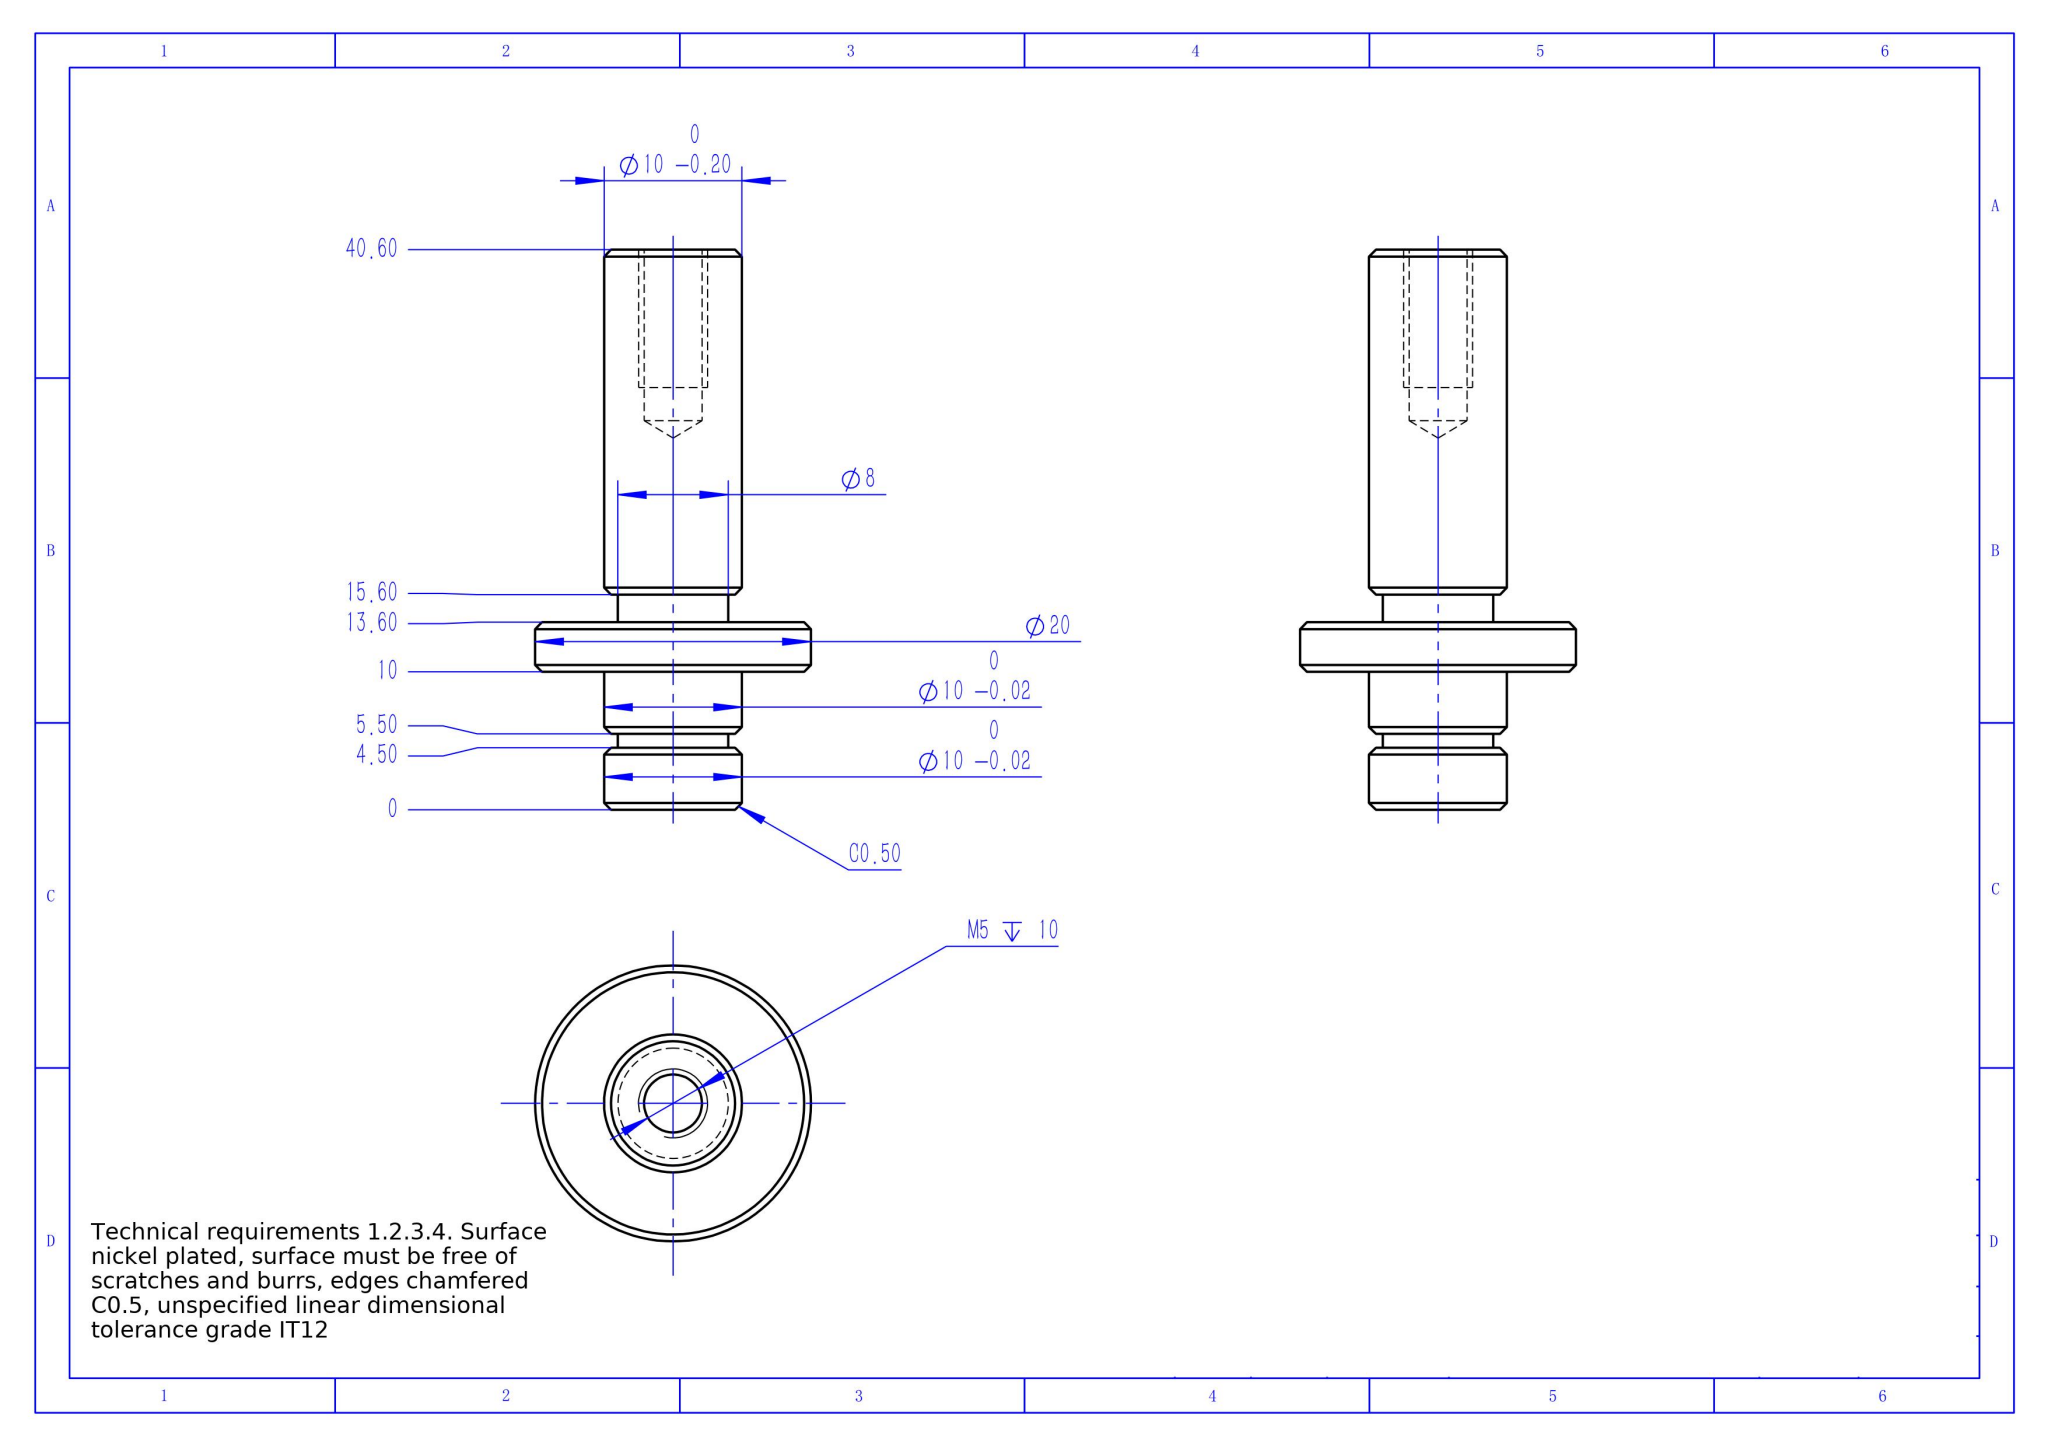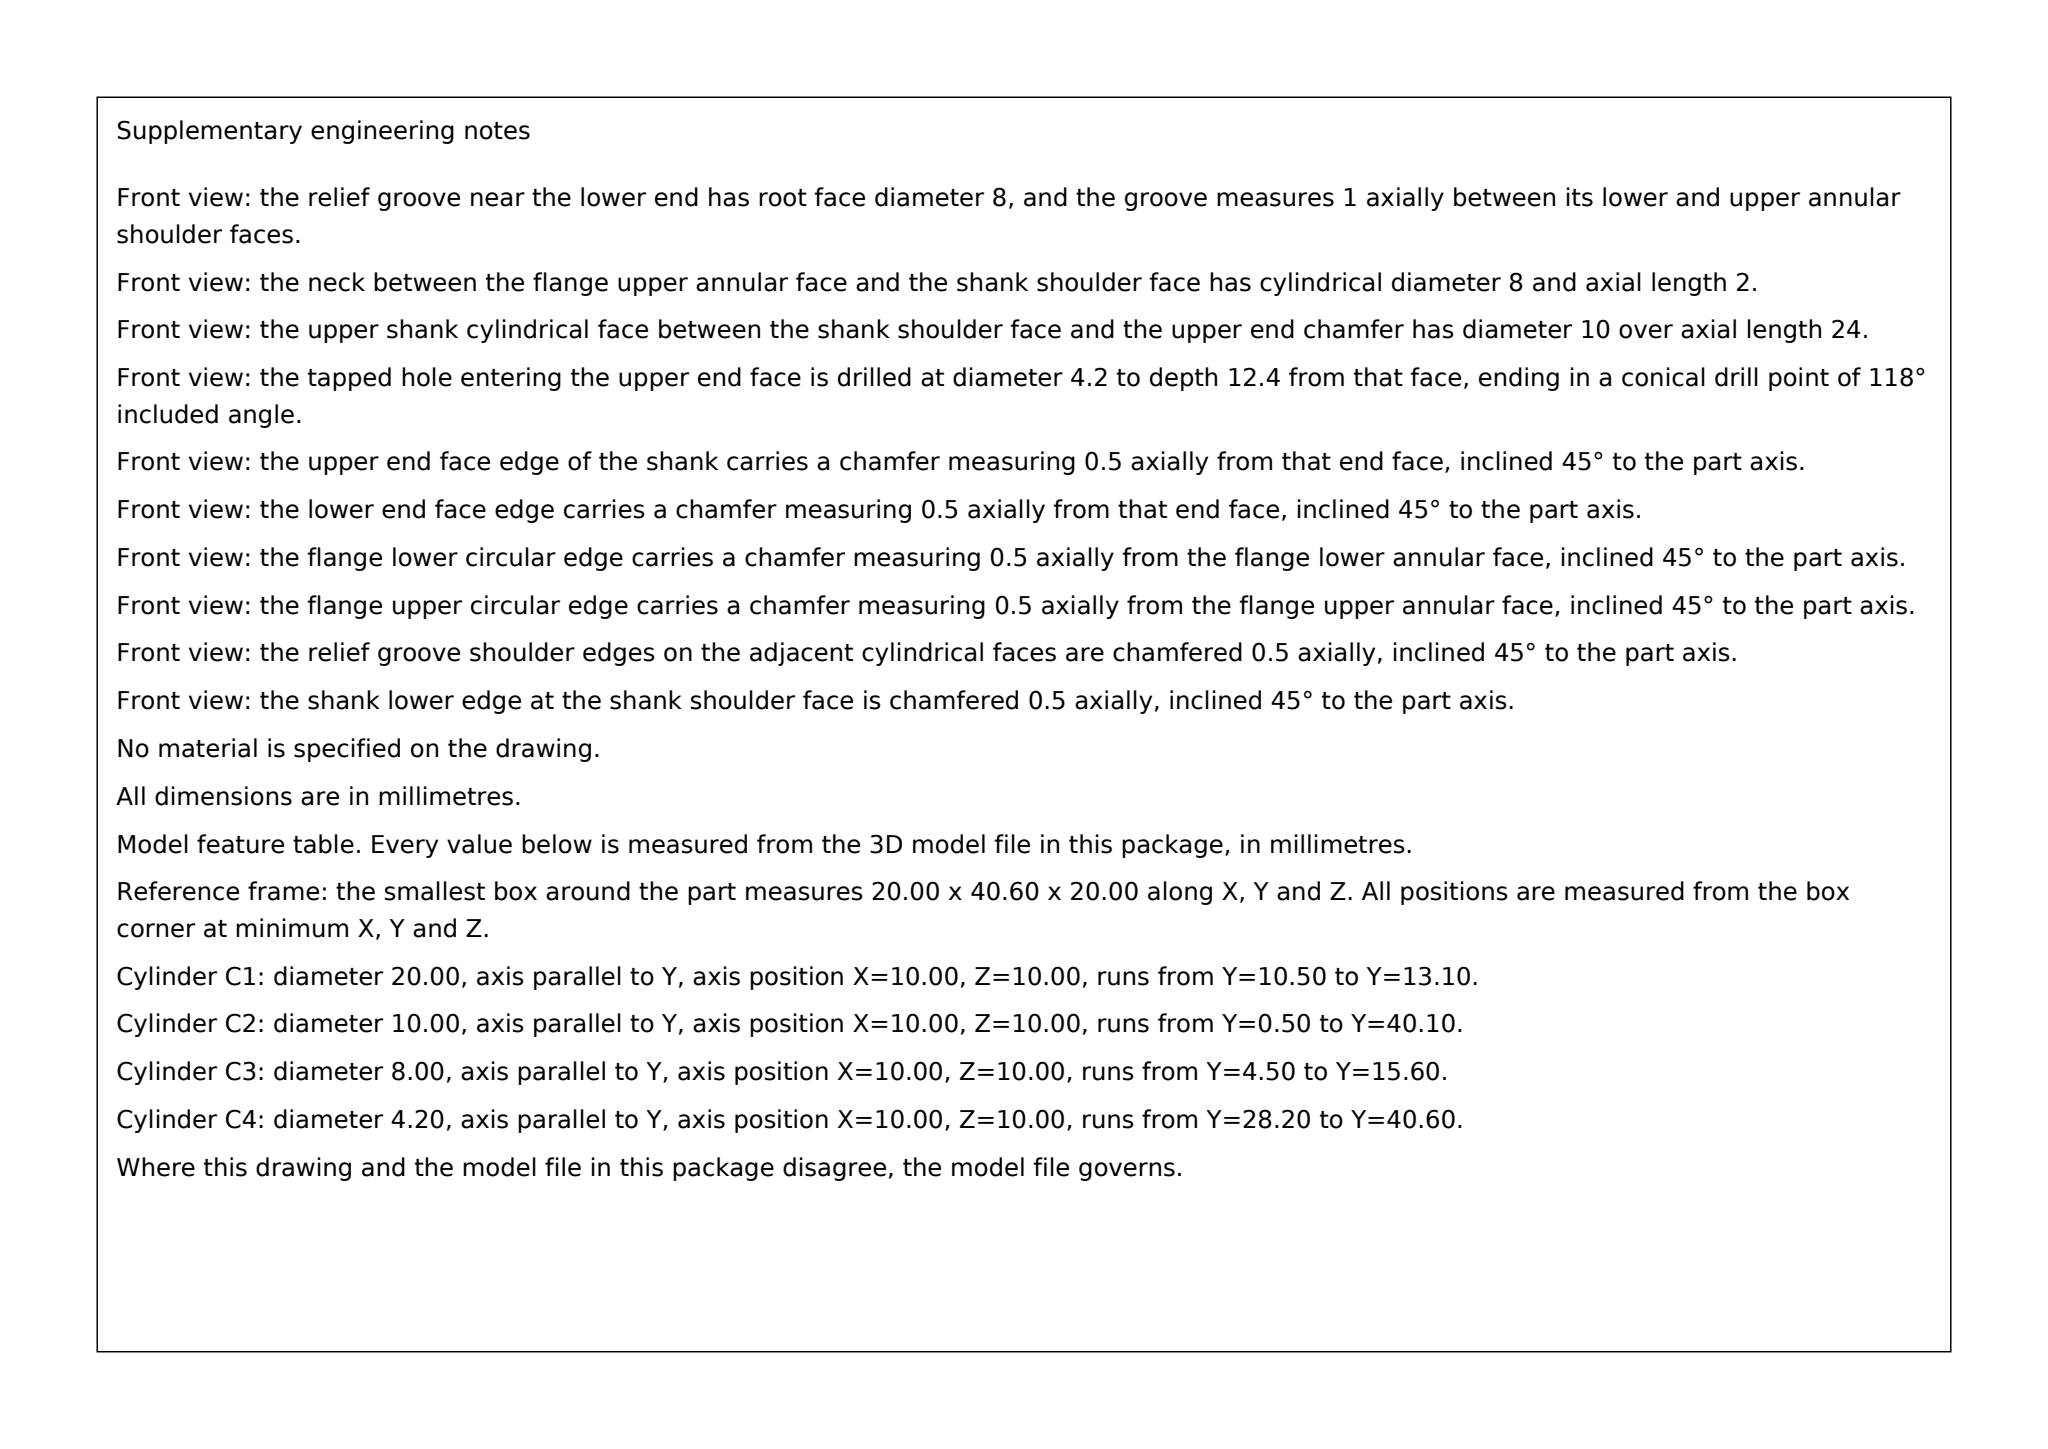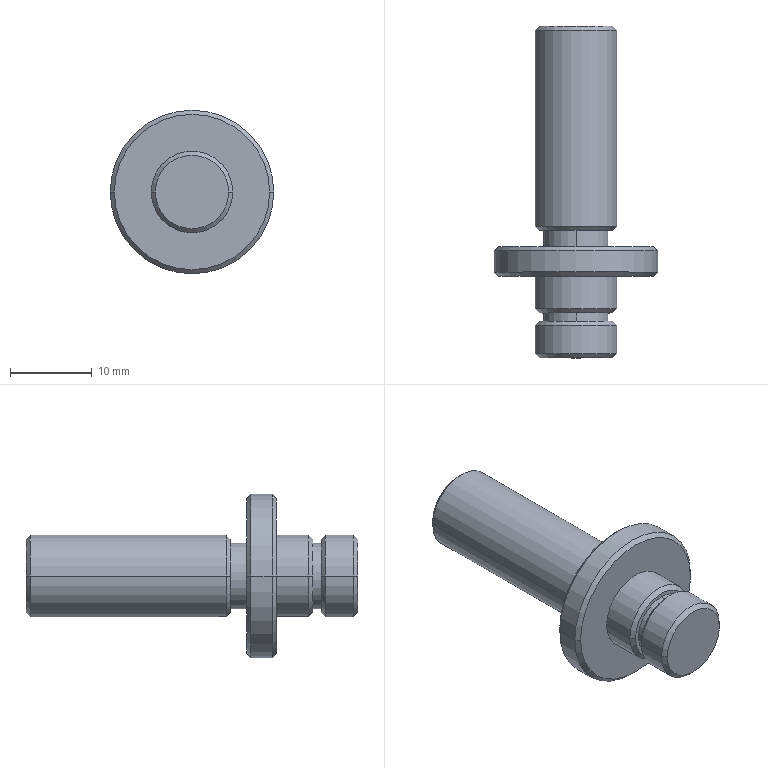Part | SolidWorks | mm | 1 solid | 37 faces | box 20 x 40.6 x 20 mm | volume 3740 mm3 | cone 16 | cylinder 14 | plane 7 | commonest cylinder face diameters 10 x6 8 x4 4.2 x2 20 x2
Drawing notes:
TAP DRILL Ø4.2 DP 12.4 FROM TOP FACE (118° PT), M5 DP 10 | from the solid: Ø4.2 cyl, axis y, length 12.4 from y=40.6 top face; 118° cone ref dia 4.2; M5 thread 10 deep
LOWER GROOVE Ø8 x 1 WIDE, 4.5 TO 5.5 FROM BOTTOM FACE | from the solid: Ø8 cyl length 1.0 between y-planes 4.5 and 5.5; y=0 bottom face datum
UPPER UNDERCUT Ø8 x 2 WIDE, 13.6 TO 15.6 FROM BOTTOM FACE | from the solid: Ø8 cyl length 2.0 between y-planes 13.6 and 15.6; existing 13.60/15.60 dims from y=0
build123d program:
from build123d import *

# Parameters (mm, degrees)
SKETCH4_W             = 1
SKETCH4_H             = 1
SKETCH4_H_2           = 2
M5_TAPPED_HOLE1_D     = 4.2
M5_TAPPED_HOLE1_DEPTH = 12.4
M5_TAPPED_HOLE1_TIP   = 1.262
CHAMFER2_SIZE         = 0.5


with BuildPart() as part:
    # Sketch1 → Revolve1 (revolve)
    with BuildSketch(Plane.XY, mode=Mode.PRIVATE) as revolve1_sk:
        Polygon((0, 0), (5, 0), (5, 10), (10, 10), (10, 13.6), (5, 13.6), (5, 40.6), (0, 40.6), align=None)
    revolve(revolve1_sk.sketch.rotate(Axis((0, 40.6, 0), (0, -1, 0)), 180), axis=Axis((0, 40.6, 0), (0, -1, 0)))

    # Sketch4 → Cut-Revolve1 (revolve, cut)
    with BuildSketch(Plane.XY, mode=Mode.PRIVATE) as cut_revolve1_sk:
        with Locations((4.5, 5)):
            Rectangle(SKETCH4_W, SKETCH4_H)
        with Locations((4.5, 14.6)):
            Rectangle(SKETCH4_W, SKETCH4_H_2)
    revolve(cut_revolve1_sk.sketch.rotate(Axis((0, 0, 0), (0, 1, 0)), 180), axis=Axis((0, 0, 0), (0, 1, 0)), mode=Mode.SUBTRACT)

    # M5 Tapped Hole1
    with Locations(Plane(origin=(0, 40.6, 0), x_dir=(1, 0, 0), z_dir=(0, 1, 0))):
        with Locations((0, 0)):
            Hole(M5_TAPPED_HOLE1_D / 2, depth=M5_TAPPED_HOLE1_DEPTH)
            with Locations((0, 0, -(M5_TAPPED_HOLE1_DEPTH + M5_TAPPED_HOLE1_TIP / 2))):  # 118° drill point
                Cone(0, M5_TAPPED_HOLE1_D / 2, M5_TAPPED_HOLE1_TIP, mode=Mode.SUBTRACT)

    # Chamfer2
    chamfer2_edges = [part.edges().sort_by_distance(p)[0] for p in [
        (5, 5.5, 0),
        (5, 4.5, 0),
        (5, 15.6, 0),
        (5, 40.6, 0),
        (10, 13.6, 0),
        (10, 10, 0),
        (5, 0, 0),
    ]]
    chamfer(chamfer2_edges, length=CHAMFER2_SIZE)


solid = part.part